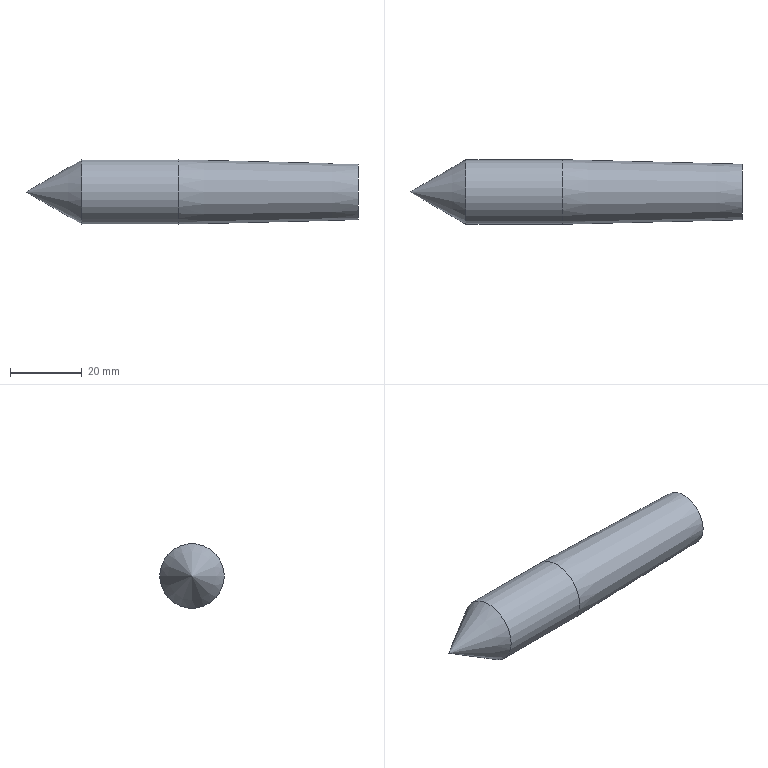Component | NX | LIVE_CENTER | 1 solid | 4 faces | box 92.59 x 18 x 18 mm | volume 19231 mm3 | cone 2 | cylinder 1 | plane 1 | commonest cylinder face diameters 18 x1
STEP:
#1=CARTESIAN_POINT('',(0.,0.,0.));
#2=DIRECTION('',(0.,0.,1.));
#3=DIRECTION('',(1.,0.,0.));
#4=AXIS2_PLACEMENT_3D('',#1,#2,#3);
#5=CARTESIAN_POINT('',(-62.588,0.,144.));
#6=VERTEX_POINT('',#5);
#7=CARTESIAN_POINT('',(-47.,9.,144.));
#8=VERTEX_POINT('',#7);
#9=CARTESIAN_POINT('',(-62.588,0.,144.));
#10=CARTESIAN_POINT('',(-47.,9.,144.));
#11=B_SPLINE_CURVE_WITH_KNOTS('',1,(#9,#10),.UNSPECIFIED.,.F.,.F.,(2,2),(-18.,0.),.PIECEWISE_BEZIER_KNOTS.);
#12=CARTESIAN_POINT('',(-47.,0.,144.));
#13=DIRECTION('',(1.,0.,0.));
#14=DIRECTION('',(0.,1.,0.));
#15=AXIS2_PLACEMENT_3D('',#12,#13,#14);
#16=CONICAL_SURFACE('',#15,9.,0.5236);
#17=CARTESIAN_POINT('',(6.283,0.));
#18=DIRECTION('',(0.,1.));
#19=VECTOR('',#18,1.);
#20=LINE('',#17,#19);
#21=(GEOMETRIC_REPRESENTATION_CONTEXT(2)PARAMETRIC_REPRESENTATION_CONTEXT()REPRESENTATION_CONTEXT('',''));
#22=DEFINITIONAL_REPRESENTATION('',(#20),#21);
#23=PCURVE('',#16,#22);
#24=CARTESIAN_POINT('',(0.,0.));
#25=DIRECTION('',(0.,1.));
#26=VECTOR('',#25,1.);
#27=LINE('',#24,#26);
#28=(GEOMETRIC_REPRESENTATION_CONTEXT(2)PARAMETRIC_REPRESENTATION_CONTEXT()REPRESENTATION_CONTEXT('',''));
#29=DEFINITIONAL_REPRESENTATION('',(#27),#28);
#30=PCURVE('',#16,#29);
#31=SEAM_CURVE('',#11,(#23,#30),.PCURVE_S1.);
#32=EDGE_CURVE('',#6,#8,#31,.T.);
#33=ORIENTED_EDGE('',*,*,#32,.T.);
#34=CARTESIAN_POINT('',(-47.,-9.,144.));
#35=VERTEX_POINT('',#34);
#36=CARTESIAN_POINT('',(-47.,0.,144.));
#37=DIRECTION('',(-1.,0.,0.));
#38=DIRECTION('',(0.,-1.,0.));
#39=AXIS2_PLACEMENT_3D('',#36,#37,#38);
#40=CIRCLE('',#39,9.);
#41=CARTESIAN_POINT('',(9.425,0.));
#42=DIRECTION('',(-1.,0.));
#43=VECTOR('',#42,1.);
#44=LINE('',#41,#43);
#45=(GEOMETRIC_REPRESENTATION_CONTEXT(2)PARAMETRIC_REPRESENTATION_CONTEXT()REPRESENTATION_CONTEXT('',''));
#46=DEFINITIONAL_REPRESENTATION('',(#44),#45);
#47=PCURVE('',#16,#46);
#48=CARTESIAN_POINT('',(31.,0.,144.));
#49=DIRECTION('',(-1.,0.,0.));
#50=DIRECTION('',(0.,-1.,0.));
#51=AXIS2_PLACEMENT_3D('',#48,#49,#50);
#52=CYLINDRICAL_SURFACE('',#51,9.);
#53=CARTESIAN_POINT('',(0.,78.));
#54=DIRECTION('',(1.,0.));
#55=VECTOR('',#54,1.);
#56=LINE('',#53,#55);
#57=(GEOMETRIC_REPRESENTATION_CONTEXT(2)PARAMETRIC_REPRESENTATION_CONTEXT()REPRESENTATION_CONTEXT('',''));
#58=DEFINITIONAL_REPRESENTATION('',(#56),#57);
#59=PCURVE('',#52,#58);
#60=SURFACE_CURVE('',#40,(#47,#59),.PCURVE_S1.);
#61=EDGE_CURVE('',#8,#35,#60,.T.);
#62=ORIENTED_EDGE('',*,*,#61,.T.);
#63=CARTESIAN_POINT('',(-47.,0.,144.));
#64=DIRECTION('',(-1.,0.,0.));
#65=DIRECTION('',(0.,-1.,0.));
#66=AXIS2_PLACEMENT_3D('',#63,#64,#65);
#67=CIRCLE('',#66,9.);
#68=CARTESIAN_POINT('',(3.142,0.));
#69=DIRECTION('',(-1.,0.));
#70=VECTOR('',#69,1.);
#71=LINE('',#68,#70);
#72=(GEOMETRIC_REPRESENTATION_CONTEXT(2)PARAMETRIC_REPRESENTATION_CONTEXT()REPRESENTATION_CONTEXT('',''));
#73=DEFINITIONAL_REPRESENTATION('',(#71),#72);
#74=PCURVE('',#16,#73);
#75=CARTESIAN_POINT('',(0.,78.));
#76=DIRECTION('',(1.,0.));
#77=VECTOR('',#76,1.);
#78=LINE('',#75,#77);
#79=(GEOMETRIC_REPRESENTATION_CONTEXT(2)PARAMETRIC_REPRESENTATION_CONTEXT()REPRESENTATION_CONTEXT('',''));
#80=DEFINITIONAL_REPRESENTATION('',(#78),#79);
#81=PCURVE('',#52,#80);
#82=SURFACE_CURVE('',#67,(#74,#81),.PCURVE_S1.);
#83=EDGE_CURVE('',#35,#8,#82,.T.);
#84=ORIENTED_EDGE('',*,*,#83,.T.);
#85=ORIENTED_EDGE('',*,*,#32,.F.);
#86=EDGE_LOOP('',(#33,#62,#84,#85));
#87=FACE_BOUND('',#86,.T.);
#88=ADVANCED_FACE('',(#87),#16,.T.);
#89=CARTESIAN_POINT('',(30.,-7.75,144.));
#90=VERTEX_POINT('',#89);
#91=CARTESIAN_POINT('',(30.,0.,144.));
#92=DIRECTION('',(-1.,0.,0.));
#93=DIRECTION('',(0.,-1.,0.));
#94=AXIS2_PLACEMENT_3D('',#91,#92,#93);
#95=CIRCLE('',#94,7.75);
#96=CARTESIAN_POINT('',(31.,0.,144.));
#97=DIRECTION('',(-1.,0.,0.));
#98=DIRECTION('',(0.,-1.,0.));
#99=AXIS2_PLACEMENT_3D('',#96,#97,#98);
#100=CONICAL_SURFACE('',#99,7.725,0.02499);
#101=CARTESIAN_POINT('',(0.,1.));
#102=DIRECTION('',(1.,0.));
#103=VECTOR('',#102,1.);
#104=LINE('',#101,#103);
#105=(GEOMETRIC_REPRESENTATION_CONTEXT(2)PARAMETRIC_REPRESENTATION_CONTEXT()REPRESENTATION_CONTEXT('',''));
#106=DEFINITIONAL_REPRESENTATION('',(#104),#105);
#107=PCURVE('',#100,#106);
#108=CARTESIAN_POINT('',(30.,15.,144.));
#109=DIRECTION('',(-1.,0.,0.));
#110=DIRECTION('',(0.,-1.,0.));
#111=AXIS2_PLACEMENT_3D('',#108,#109,#110);
#112=PLANE('',#111);
#113=CARTESIAN_POINT('',(15.,0.));
#114=DIRECTION('',(1.,0.));
#115=AXIS2_PLACEMENT_2D('',#113,#114);
#116=CIRCLE('',#115,7.75);
#117=(GEOMETRIC_REPRESENTATION_CONTEXT(2)PARAMETRIC_REPRESENTATION_CONTEXT()REPRESENTATION_CONTEXT('',''));
#118=DEFINITIONAL_REPRESENTATION('',(#116),#117);
#119=PCURVE('',#112,#118);
#120=SURFACE_CURVE('',#95,(#107,#119),.PCURVE_S1.);
#121=EDGE_CURVE('',#90,#90,#120,.T.);
#122=ORIENTED_EDGE('',*,*,#121,.T.);
#123=CARTESIAN_POINT('',(-20.,-9.,144.));
#124=VERTEX_POINT('',#123);
#125=CARTESIAN_POINT('',(30.,-7.75,144.));
#126=CARTESIAN_POINT('',(-20.,-9.,144.));
#127=B_SPLINE_CURVE_WITH_KNOTS('',1,(#125,#126),.UNSPECIFIED.,.F.,.F.,(2,2),(1.,51.016),.PIECEWISE_BEZIER_KNOTS.);
#128=CARTESIAN_POINT('',(6.283,0.));
#129=DIRECTION('',(0.,1.));
#130=VECTOR('',#129,1.);
#131=LINE('',#128,#130);
#132=(GEOMETRIC_REPRESENTATION_CONTEXT(2)PARAMETRIC_REPRESENTATION_CONTEXT()REPRESENTATION_CONTEXT('',''));
#133=DEFINITIONAL_REPRESENTATION('',(#131),#132);
#134=PCURVE('',#100,#133);
#135=CARTESIAN_POINT('',(0.,0.));
#136=DIRECTION('',(0.,1.));
#137=VECTOR('',#136,1.);
#138=LINE('',#135,#137);
#139=(GEOMETRIC_REPRESENTATION_CONTEXT(2)PARAMETRIC_REPRESENTATION_CONTEXT()REPRESENTATION_CONTEXT('',''));
#140=DEFINITIONAL_REPRESENTATION('',(#138),#139);
#141=PCURVE('',#100,#140);
#142=SEAM_CURVE('',#127,(#134,#141),.PCURVE_S1.);
#143=EDGE_CURVE('',#90,#124,#142,.T.);
#144=ORIENTED_EDGE('',*,*,#143,.T.);
#145=CARTESIAN_POINT('',(-20.,0.,144.));
#146=DIRECTION('',(-1.,0.,0.));
#147=DIRECTION('',(0.,-1.,0.));
#148=AXIS2_PLACEMENT_3D('',#145,#146,#147);
#149=CIRCLE('',#148,9.);
#150=CARTESIAN_POINT('',(0.,51.));
#151=DIRECTION('',(1.,0.));
#152=VECTOR('',#151,1.);
#153=LINE('',#150,#152);
#154=(GEOMETRIC_REPRESENTATION_CONTEXT(2)PARAMETRIC_REPRESENTATION_CONTEXT()REPRESENTATION_CONTEXT('',''));
#155=DEFINITIONAL_REPRESENTATION('',(#153),#154);
#156=PCURVE('',#100,#155);
#157=CARTESIAN_POINT('',(0.,51.));
#158=DIRECTION('',(1.,0.));
#159=VECTOR('',#158,1.);
#160=LINE('',#157,#159);
#161=(GEOMETRIC_REPRESENTATION_CONTEXT(2)PARAMETRIC_REPRESENTATION_CONTEXT()REPRESENTATION_CONTEXT('',''));
#162=DEFINITIONAL_REPRESENTATION('',(#160),#161);
#163=PCURVE('',#52,#162);
#164=SURFACE_CURVE('',#149,(#156,#163),.PCURVE_S1.);
#165=EDGE_CURVE('',#124,#124,#164,.T.);
#166=ORIENTED_EDGE('',*,*,#165,.F.);
#167=ORIENTED_EDGE('',*,*,#143,.F.);
#168=EDGE_LOOP('',(#122,#144,#166,#167));
#169=FACE_BOUND('',#168,.T.);
#170=ADVANCED_FACE('',(#169),#100,.T.);
#171=ORIENTED_EDGE('',*,*,#83,.F.);
#172=CARTESIAN_POINT('',(-20.,-9.,144.));
#173=CARTESIAN_POINT('',(-47.,-9.,144.));
#174=B_SPLINE_CURVE_WITH_KNOTS('',1,(#172,#173),.UNSPECIFIED.,.F.,.F.,(2,2),(51.,78.),.PIECEWISE_BEZIER_KNOTS.);
#175=CARTESIAN_POINT('',(0.,0.));
#176=DIRECTION('',(0.,1.));
#177=VECTOR('',#176,1.);
#178=LINE('',#175,#177);
#179=(GEOMETRIC_REPRESENTATION_CONTEXT(2)PARAMETRIC_REPRESENTATION_CONTEXT()REPRESENTATION_CONTEXT('',''));
#180=DEFINITIONAL_REPRESENTATION('',(#178),#179);
#181=PCURVE('',#52,#180);
#182=CARTESIAN_POINT('',(6.283,0.));
#183=DIRECTION('',(0.,1.));
#184=VECTOR('',#183,1.);
#185=LINE('',#182,#184);
#186=(GEOMETRIC_REPRESENTATION_CONTEXT(2)PARAMETRIC_REPRESENTATION_CONTEXT()REPRESENTATION_CONTEXT('',''));
#187=DEFINITIONAL_REPRESENTATION('',(#185),#186);
#188=PCURVE('',#52,#187);
#189=SEAM_CURVE('',#174,(#181,#188),.PCURVE_S1.);
#190=EDGE_CURVE('',#124,#35,#189,.T.);
#191=ORIENTED_EDGE('',*,*,#190,.F.);
#192=ORIENTED_EDGE('',*,*,#165,.T.);
#193=ORIENTED_EDGE('',*,*,#190,.T.);
#194=ORIENTED_EDGE('',*,*,#61,.F.);
#195=EDGE_LOOP('',(#171,#191,#192,#193,#194));
#196=FACE_BOUND('',#195,.T.);
#197=ADVANCED_FACE('',(#196),#52,.T.);
#198=ORIENTED_EDGE('',*,*,#121,.F.);
#199=EDGE_LOOP('',(#198));
#200=FACE_BOUND('',#199,.T.);
#201=ADVANCED_FACE('',(#200),#112,.F.);
#202=CLOSED_SHELL('',(#88,#170,#197,#201));
#203=MANIFOLD_SOLID_BREP('',#202);
#204=(LENGTH_UNIT()NAMED_UNIT(*)SI_UNIT(.MILLI.,.METRE.));
#205=UNCERTAINTY_MEASURE_WITH_UNIT(LENGTH_MEASURE(0.00001),#204,'','');
#206=(NAMED_UNIT(*)PLANE_ANGLE_UNIT()SI_UNIT($,.RADIAN.));
#207=(NAMED_UNIT(*)SI_UNIT($,.STERADIAN.)SOLID_ANGLE_UNIT());
#208=(GEOMETRIC_REPRESENTATION_CONTEXT(3)GLOBAL_UNCERTAINTY_ASSIGNED_CONTEXT((#205))GLOBAL_UNIT_ASSIGNED_CONTEXT((#204,#206,#207))REPRESENTATION_CONTEXT('',''));
#209=ADVANCED_BREP_SHAPE_REPRESENTATION('',(#4,#203),#208);